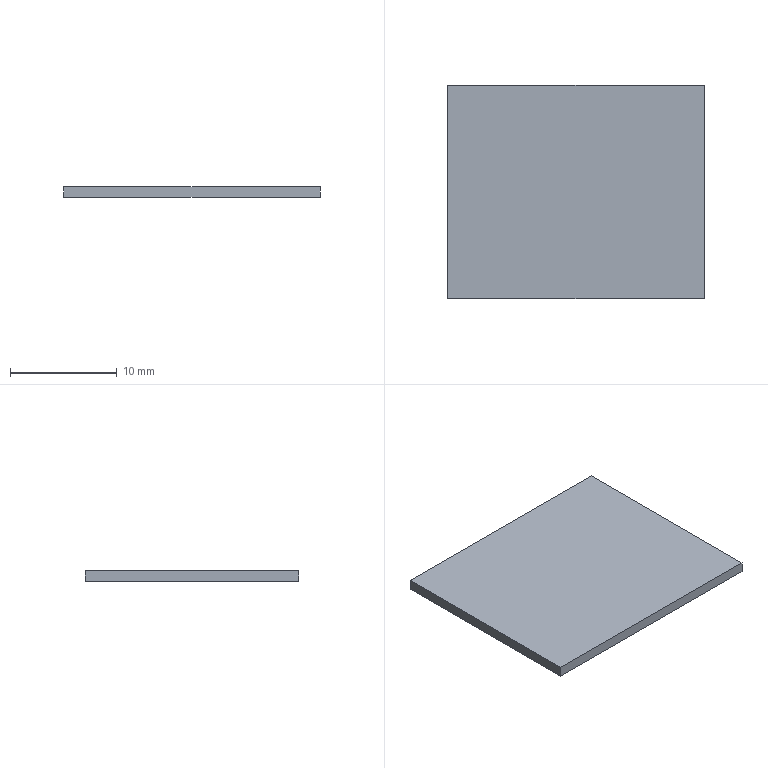Component | SolidWorks | OuterBagExpansionSheetMetalSideSeal-1 | 1 solid | 6 faces | box 24 x 20 x 1 mm | volume 480 mm3 | plane 6
build123d program:
from build123d import *

# Parameters (mm, degrees)
SKETCH2_W           = 20
SKETCH2_H           = 24
BOSS_EXTRUDE1_DEPTH = 1


with BuildPart() as part:
    # Sketch2 → Boss-Extrude1 (new body)
    with BuildSketch(Plane.XY):
        with Locations((9.169, -12)):
            Rectangle(SKETCH2_W, SKETCH2_H)
    extrude(amount=BOSS_EXTRUDE1_DEPTH)


solid = part.part

# Placed as in the assembly
solid = solid.moved(Location((-550.446, 3.257, 413.468), (0, 0, 90)))